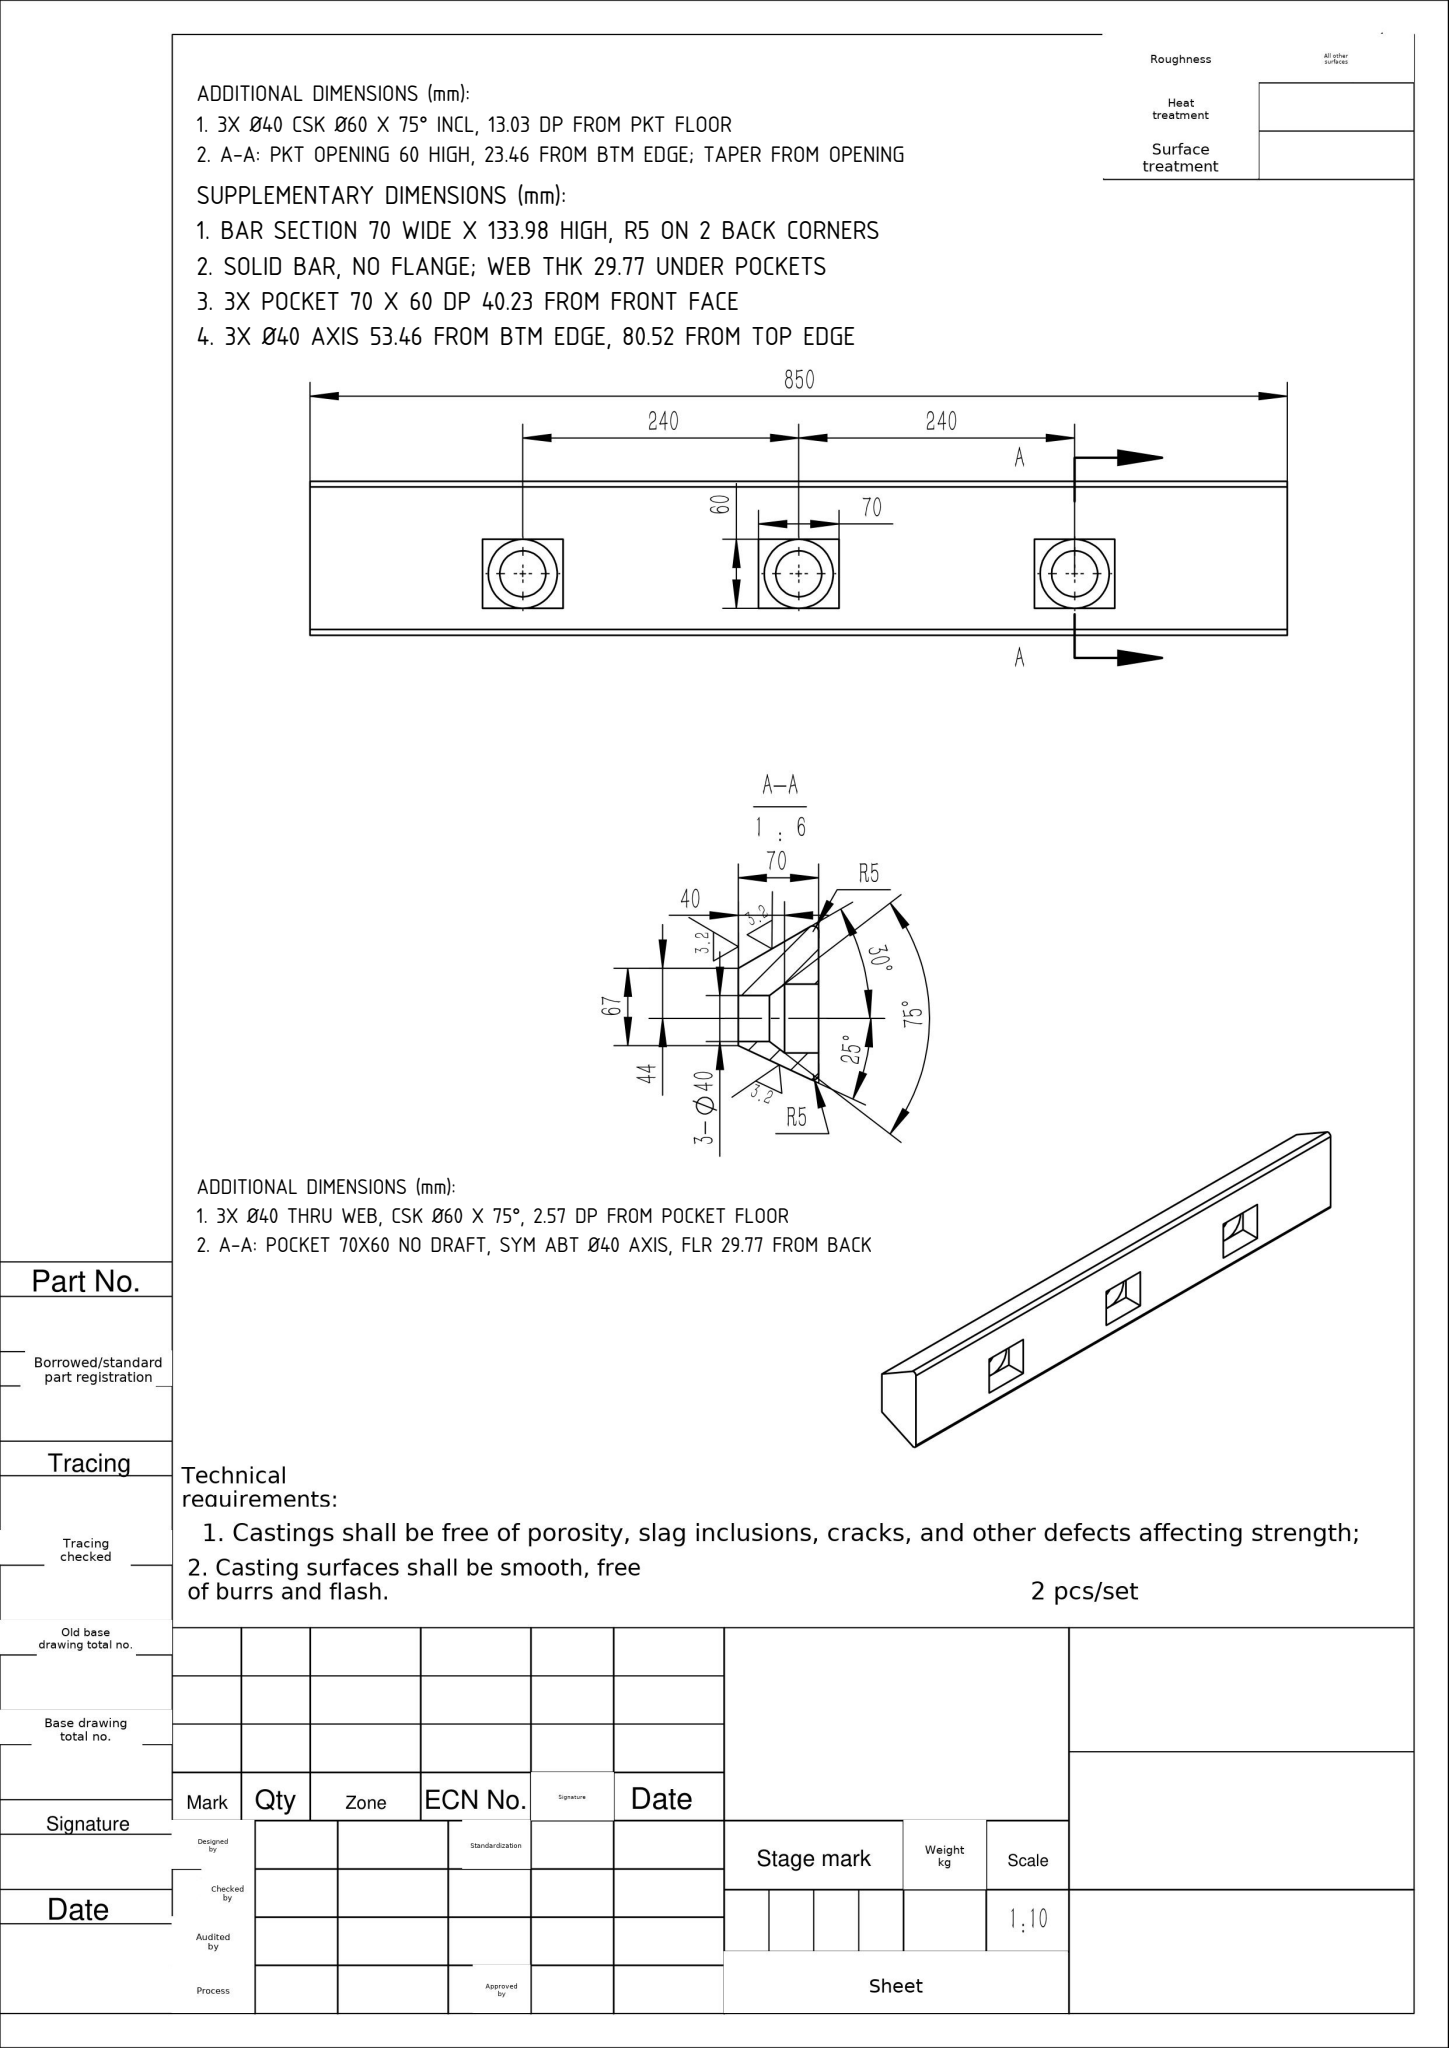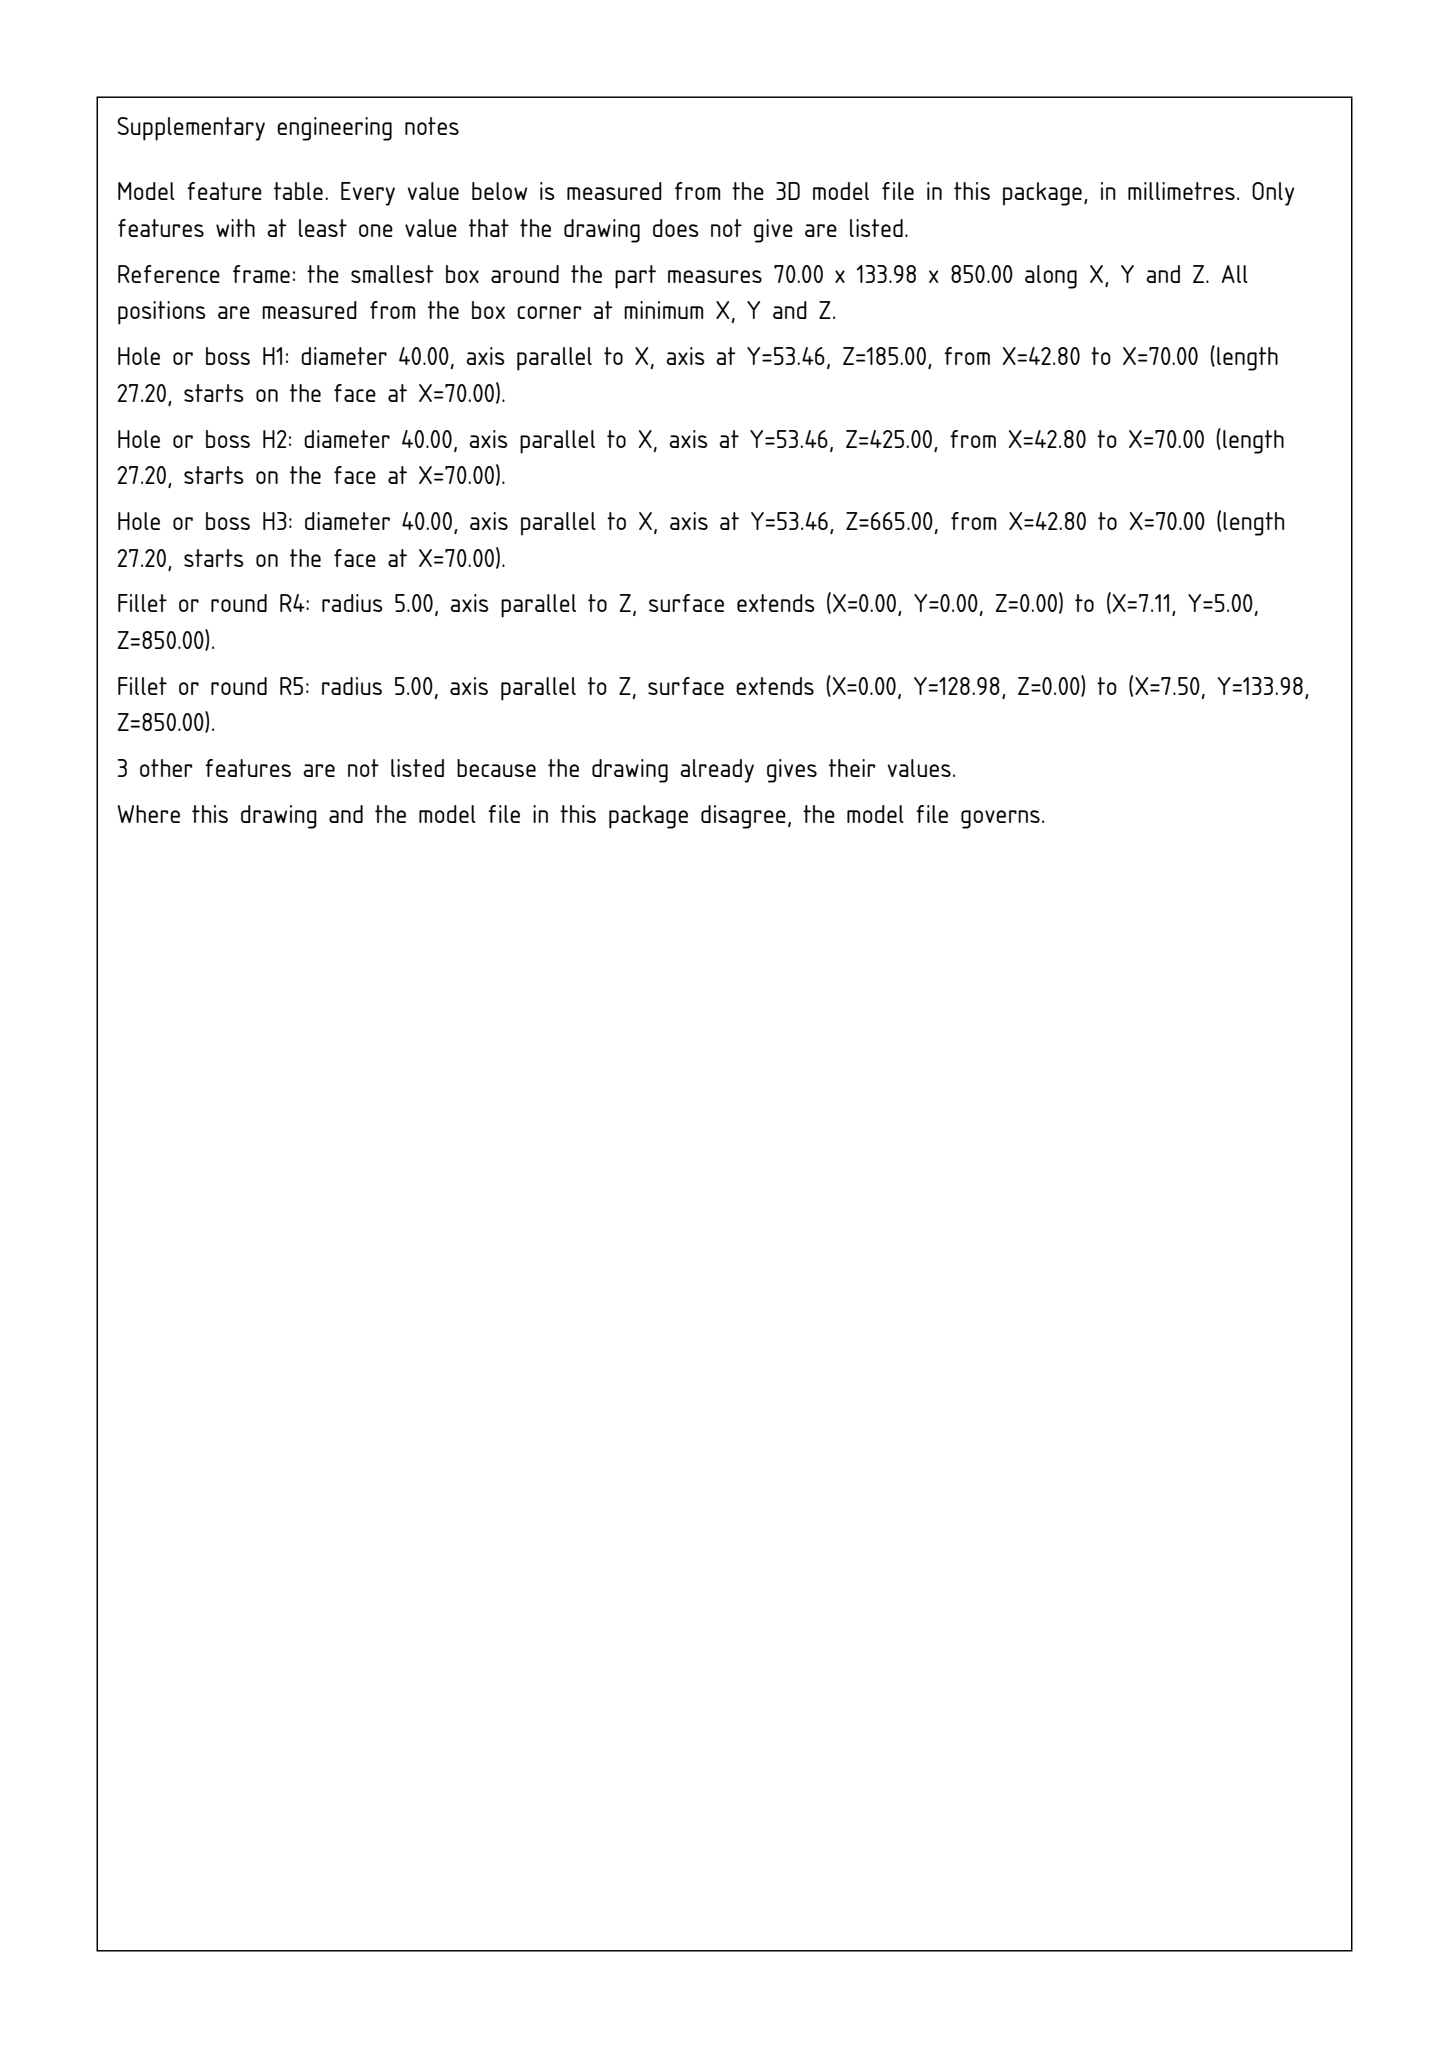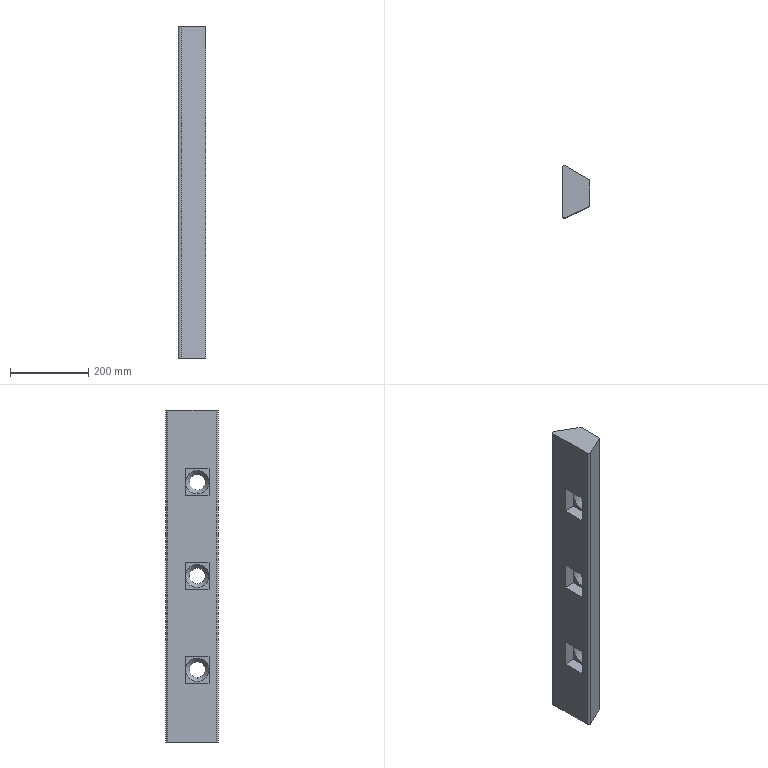Part | SolidWorks | mm | 1 solid | 38 faces | box 70 x 133.98 x 850 mm | volume 5603906 mm3 | plane 24 | cylinder 8 | cone 6 | commonest cylinder face diameters 40 x6 10 x2
build123d program:
from build123d import *

# Parameters (mm, degrees)
SKETCH1_W            = 130
SKETCH1_H            = 300
BOSS_EXTRUDE1_DEPTH  = 425
SKETCH10_OUTSIDE_W   = 1034.142
SKETCH10_OUTSIDE_H   = 484.142
SKETCH10_OUTSIDE_W_2 = 870
SKETCH10_OUTSIDE_H_2 = 249.778
CUT_EXTRUDE7_DEPTH   = 195
SKETCH14_W           = 70
SKETCH14_H           = 60
CUT_EXTRUDE8_DEPTH   = 120
SKETCH15_R           = 20
CUT_EXTRUDE9_DEPTH   = 100
SKETCH16_W           = 22.8
SKETCH16_H           = 249.778
CUT_EXTRUDE10_DEPTH  = 905.913
SKETCH17_W           = 27.2
SKETCH17_H           = 249.778
CUT_EXTRUDE11_DEPTH  = 902.92
LPATTERN1_COUNT      = 3
LPATTERN1_PITCH      = 240
SKETCH18_OUTSIDE_W   = 259.908
SKETCH18_OUTSIDE_H   = 429.687
CUT_EXTRUDE12_DEPTH  = 902.92
SKETCH19_W           = 10
SKETCH19_H           = 102.156
CUT_EXTRUDE13_DEPTH  = 898.104
FILLET2_R            = 5


with BuildPart() as part:
    # Sketch1 → Boss-Extrude1 (new, symmetric)
    with BuildSketch(Plane.XY):
        with Locations((65, 150)):
            Rectangle(SKETCH1_W, SKETCH1_H)
    extrude(amount=BOSS_EXTRUDE1_DEPTH, both=True)

    # Sketch10 outside → Cut-Extrude7 (cut)
    with BuildSketch(Plane.ZY):
        with Locations((0, 150)):
            Rectangle(SKETCH10_OUTSIDE_W, SKETCH10_OUTSIDE_H)
        with Locations((0, 157.011)):
            Rectangle(SKETCH10_OUTSIDE_W_2, SKETCH10_OUTSIDE_H_2, mode=Mode.SUBTRACT)
    extrude(amount=-CUT_EXTRUDE7_DEPTH, mode=Mode.SUBTRACT)

    # Sketch13 → Cut-Revolve1 (revolve, cut)
    with BuildSketch(Plane(origin=(0, 0, -240), x_dir=(-1, 0, 0), z_dir=(0, 0, -1)), mode=Mode.PRIVATE) as cut_revolve1_sk:
        Polygon((-70, 181.901), (-70, 201.901), (-56.968, 211.901), (-56.968, 181.901), align=None)
    cut_revolve1 = revolve(cut_revolve1_sk.sketch.rotate(Axis((174.363, 181.901, -240), (-1, 0, 0)), 90), axis=Axis((174.363, 181.901, -240), (-1, 0, 0)), mode=Mode.SUBTRACT)

    # Sketch14 → Cut-Extrude8 (cut)
    with BuildSketch(Plane(origin=(56.968, 0, 0), x_dir=(0, 0, -1), z_dir=(1, 0, 0))):
        with Locations((240, 181.901)):
            Rectangle(SKETCH14_W, SKETCH14_H)
    cut_extrude8 = extrude(amount=-CUT_EXTRUDE8_DEPTH, mode=Mode.SUBTRACT)

    # Sketch15 → Cut-Extrude9 (cut)
    with BuildSketch(Plane.ZY.offset(-70)):
        with Locations((-240, 181.901)):
            Circle(SKETCH15_R)
    cut_extrude9 = extrude(amount=-CUT_EXTRUDE9_DEPTH, mode=Mode.SUBTRACT)

    # Sketch16 → Cut-Extrude10 (cut, through all)
    with BuildSketch(Plane(origin=(0, 0, -425), x_dir=(-1, 0, 0), z_dir=(0, 0, -1))):
        with Locations((-118.6, 157.011)):
            Rectangle(SKETCH16_W, SKETCH16_H)
    extrude(amount=-CUT_EXTRUDE10_DEPTH, mode=Mode.SUBTRACT)

    # Sketch17 → Cut-Extrude11 (cut, through all)
    with BuildSketch(Plane(origin=(0, 0, -425), x_dir=(-1, 0, 0), z_dir=(0, 0, -1))):
        with Locations((-13.6, 157.011)):
            Rectangle(SKETCH17_W, SKETCH17_H)
    extrude(amount=-CUT_EXTRUDE11_DEPTH, mode=Mode.SUBTRACT)

    # LPattern1: Cut-Revolve1, Cut-Extrude8, Cut-Extrude9 ×3
    with Locations(*[(0, 0, i * LPATTERN1_PITCH) for i in range(1, LPATTERN1_COUNT)]):
        add(cut_revolve1, mode=Mode.SUBTRACT)
        add(cut_extrude8, mode=Mode.SUBTRACT)
        add(cut_extrude9, mode=Mode.SUBTRACT)

    # Sketch18 outside → Cut-Extrude12 (cut, through all)
    with BuildSketch(Plane(origin=(0, 0, -425), x_dir=(-1, 0, 0), z_dir=(0, 0, -1))):
        with Locations((-67.2, 157.012)):
            Rectangle(SKETCH18_OUTSIDE_W, SKETCH18_OUTSIDE_H)
        Polygon((-107.2, 219.901), (-27.2, 266.089), (-27.2, 125.596), (-107.2, 162.901), align=None, mode=Mode.SUBTRACT)
    extrude(amount=-CUT_EXTRUDE12_DEPTH, mode=Mode.SUBTRACT)

    # Sketch19 → Cut-Extrude13 (cut, through all)
    with BuildSketch(Plane(origin=(0, 0, -425), x_dir=(-1, 0, 0), z_dir=(0, 0, -1))):
        with Locations((-102.2, 193.037)):
            Rectangle(SKETCH19_W, SKETCH19_H)
    extrude(amount=-CUT_EXTRUDE13_DEPTH, mode=Mode.SUBTRACT)

    # Fillet2
    fillet2_edges = [part.edges().sort_by_distance(p)[0] for p in [
        (27.2, 125.596, 0),
        (27.2, 266.089, 0),
    ]]
    fillet(fillet2_edges, radius=FILLET2_R)


solid = part.part